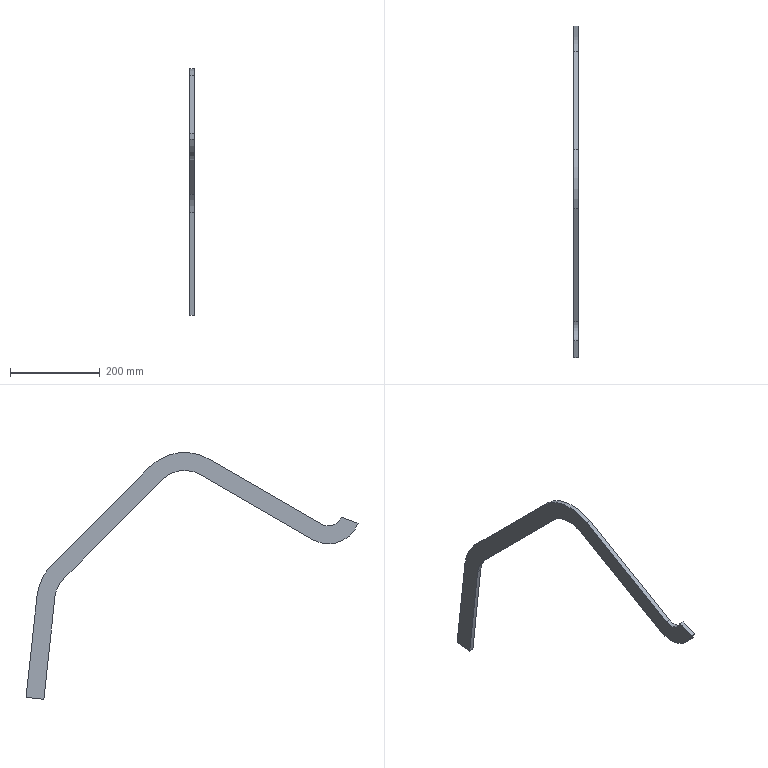Component | SolidWorks | Rebro sipke-3-109 | 1 solid | 16 faces | box 10 x 740.76 x 550.54 mm | volume 438581 mm3 | plane 10 | cylinder 6 | commonest cylinder face diameters 140 x3 220 x2 60 x1
build123d program:
from build123d import *

# Parameters (mm, degrees)
BOSS_EXTRUDE1_DEPTH = 10


with BuildPart() as part:
    # Sketch1 → Boss-Extrude1 (new body)
    with BuildSketch(Plane.XY):
        with BuildLine():
            Line((626.269, -76.361), (701.294, 203.766))
            ThreePointArc((701.294, 203.766), (739.32, 249.094), (798.487, 249.101))
            Line((798.487, 249.101), (781.586, 212.847))
            ThreePointArc((781.586, 212.847), (756.229, 212.844), (739.932, 193.418))
            Line((739.932, 193.418), (664.907, -86.71))
            ThreePointArc((664.907, -86.71), (625.621, -145.517), (558.652, -168.252))
            Line((558.652, -168.252), (248.065, -168.252))
            ThreePointArc((248.065, -168.252), (211.537, -162.01), (179.154, -143.991))
            Line((179.154, -143.991), (0, 0))
            Line((0, 0), (25.059, 31.178))
            Line((25.059, 31.178), (204.213, -112.813))
            ThreePointArc((204.213, -112.813), (224.82, -124.279), (248.065, -128.252))
            Line((248.065, -128.252), (558.652, -128.252))
            ThreePointArc((558.652, -128.252), (601.269, -113.784), (626.269, -76.361))
        make_face()
    extrude(amount=-BOSS_EXTRUDE1_DEPTH)


solid = part.part

# Placed as in the assembly
solid = solid.moved(Location((-91.6, -141.455, -674.126), (-135, 90, 0)))
STEP:
#1=COLOUR_RGB('',0.7922,0.8196,0.9333);
#2=FILL_AREA_STYLE_COLOUR('',#1);
#3=FILL_AREA_STYLE('',(#2));
#4=SURFACE_STYLE_FILL_AREA(#3);
#5=SURFACE_SIDE_STYLE('',(#4));
#6=SURFACE_STYLE_USAGE(.BOTH.,#5);
#7=PRESENTATION_STYLE_ASSIGNMENT((#6));
#8=CARTESIAN_POINT('',(-3.606,-34.733,-11.246));
#9=VERTEX_POINT('',#8);
#10=CARTESIAN_POINT('',(-3.606,-30.765,-12.69));
#11=VERTEX_POINT('',#10);
#12=CARTESIAN_POINT('',(-3.606,-32.143,-10.303));
#13=DIRECTION('',(1.,-0.,-0.));
#14=DIRECTION('',(0.,-0.7071,0.7071));
#15=AXIS2_PLACEMENT_3D('',#12,#13,#14);
#16=CIRCLE('',#15,2.756);
#17=EDGE_CURVE('',#9,#11,#16,.T.);
#18=ORIENTED_EDGE('',*,*,#17,.F.);
#19=CARTESIAN_POINT('',(-4.,-34.733,-11.246));
#20=VERTEX_POINT('',#19);
#21=CARTESIAN_POINT('',(-4.,-34.733,-11.246));
#22=DIRECTION('',(1.,-0.,-0.));
#23=VECTOR('',#22,39.37);
#24=LINE('',#21,#23);
#25=EDGE_CURVE('',#20,#9,#24,.T.);
#26=ORIENTED_EDGE('',*,*,#25,.F.);
#27=CARTESIAN_POINT('',(-4.,-30.765,-12.69));
#28=VERTEX_POINT('',#27);
#29=CARTESIAN_POINT('',(-4.,-32.143,-10.303));
#30=DIRECTION('',(1.,-0.,-0.));
#31=DIRECTION('',(0.,-0.7071,0.7071));
#32=AXIS2_PLACEMENT_3D('',#29,#30,#31);
#33=CIRCLE('',#32,2.756);
#34=EDGE_CURVE('',#20,#28,#33,.T.);
#35=ORIENTED_EDGE('',*,*,#34,.T.);
#36=CARTESIAN_POINT('',(-4.,-30.765,-12.69));
#37=DIRECTION('',(1.,-0.,-0.));
#38=VECTOR('',#37,39.37);
#39=LINE('',#36,#38);
#40=EDGE_CURVE('',#28,#11,#39,.T.);
#41=ORIENTED_EDGE('',*,*,#40,.T.);
#42=EDGE_LOOP('',(#18,#26,#35,#41));
#43=FACE_OUTER_BOUND('',#42,.T.);
#44=CARTESIAN_POINT('',(-4.,-32.143,-10.303));
#45=DIRECTION('',(1.,-0.,-0.));
#46=DIRECTION('',(0.,-0.7071,0.7071));
#47=AXIS2_PLACEMENT_3D('',#44,#45,#46);
#48=CYLINDRICAL_SURFACE('',#47,2.756);
#49=ADVANCED_FACE('',(#43),#48,.T.);
#50=CARTESIAN_POINT('',(-3.606,-33.253,-10.707));
#51=VERTEX_POINT('',#50);
#52=CARTESIAN_POINT('',(-3.606,-33.253,-10.707));
#53=DIRECTION('',(-0.,-0.9397,-0.3421));
#54=VECTOR('',#53,39.37);
#55=LINE('',#52,#54);
#56=EDGE_CURVE('',#51,#9,#55,.T.);
#57=ORIENTED_EDGE('',*,*,#56,.F.);
#58=CARTESIAN_POINT('',(-4.,-33.253,-10.707));
#59=VERTEX_POINT('',#58);
#60=CARTESIAN_POINT('',(-4.,-33.253,-10.707));
#61=DIRECTION('',(1.,-0.,-0.));
#62=VECTOR('',#61,39.37);
#63=LINE('',#60,#62);
#64=EDGE_CURVE('',#59,#51,#63,.T.);
#65=ORIENTED_EDGE('',*,*,#64,.F.);
#66=CARTESIAN_POINT('',(-4.,-33.253,-10.707));
#67=DIRECTION('',(-0.,-0.9397,-0.3421));
#68=VECTOR('',#67,39.37);
#69=LINE('',#66,#68);
#70=EDGE_CURVE('',#59,#20,#69,.T.);
#71=ORIENTED_EDGE('',*,*,#70,.T.);
#72=ORIENTED_EDGE('',*,*,#25,.T.);
#73=EDGE_LOOP('',(#57,#65,#71,#72));
#74=FACE_OUTER_BOUND('',#73,.T.);
#75=CARTESIAN_POINT('',(-4.,-33.253,-10.707));
#76=DIRECTION('',(0.,-0.3421,0.9397));
#77=DIRECTION('',(-0.,-0.9397,-0.3421));
#78=AXIS2_PLACEMENT_3D('',#75,#76,#77);
#79=PLANE('',#78);
#80=ADVANCED_FACE('',(#74),#79,.T.);
#81=CARTESIAN_POINT('',(-3.606,-31.552,-11.326));
#82=VERTEX_POINT('',#81);
#83=CARTESIAN_POINT('',(-3.606,-32.143,-10.303));
#84=DIRECTION('',(-1.,0.,0.));
#85=DIRECTION('',(0.,-0.7071,0.7071));
#86=AXIS2_PLACEMENT_3D('',#83,#84,#85);
#87=CIRCLE('',#86,1.181);
#88=EDGE_CURVE('',#82,#51,#87,.T.);
#89=ORIENTED_EDGE('',*,*,#88,.F.);
#90=CARTESIAN_POINT('',(-4.,-31.552,-11.326));
#91=VERTEX_POINT('',#90);
#92=CARTESIAN_POINT('',(-4.,-31.552,-11.326));
#93=DIRECTION('',(1.,-0.,-0.));
#94=VECTOR('',#93,39.37);
#95=LINE('',#92,#94);
#96=EDGE_CURVE('',#91,#82,#95,.T.);
#97=ORIENTED_EDGE('',*,*,#96,.F.);
#98=CARTESIAN_POINT('',(-4.,-32.143,-10.303));
#99=DIRECTION('',(-1.,0.,0.));
#100=DIRECTION('',(0.,-0.7071,0.7071));
#101=AXIS2_PLACEMENT_3D('',#98,#99,#100);
#102=CIRCLE('',#101,1.181);
#103=EDGE_CURVE('',#91,#59,#102,.T.);
#104=ORIENTED_EDGE('',*,*,#103,.T.);
#105=ORIENTED_EDGE('',*,*,#64,.T.);
#106=EDGE_LOOP('',(#89,#97,#104,#105));
#107=FACE_OUTER_BOUND('',#106,.T.);
#108=CARTESIAN_POINT('',(-4.,-32.143,-10.303));
#109=DIRECTION('',(1.,-0.,-0.));
#110=DIRECTION('',(0.,-0.7071,0.7071));
#111=AXIS2_PLACEMENT_3D('',#108,#109,#110);
#112=CYLINDRICAL_SURFACE('',#111,1.181);
#113=ADVANCED_FACE('',(#107),#112,.F.);
#114=CARTESIAN_POINT('',(-3.606,-21.665,-5.616));
#115=VERTEX_POINT('',#114);
#116=CARTESIAN_POINT('',(-3.606,-21.665,-5.616));
#117=DIRECTION('',(-0.,-0.866,-0.5001));
#118=VECTOR('',#117,39.37);
#119=LINE('',#116,#118);
#120=EDGE_CURVE('',#115,#82,#119,.T.);
#121=ORIENTED_EDGE('',*,*,#120,.F.);
#122=CARTESIAN_POINT('',(-4.,-21.665,-5.616));
#123=VERTEX_POINT('',#122);
#124=CARTESIAN_POINT('',(-4.,-21.665,-5.616));
#125=DIRECTION('',(1.,-0.,-0.));
#126=VECTOR('',#125,39.37);
#127=LINE('',#124,#126);
#128=EDGE_CURVE('',#123,#115,#127,.T.);
#129=ORIENTED_EDGE('',*,*,#128,.F.);
#130=CARTESIAN_POINT('',(-4.,-21.665,-5.616));
#131=DIRECTION('',(-0.,-0.866,-0.5001));
#132=VECTOR('',#131,39.37);
#133=LINE('',#130,#132);
#134=EDGE_CURVE('',#123,#91,#133,.T.);
#135=ORIENTED_EDGE('',*,*,#134,.T.);
#136=ORIENTED_EDGE('',*,*,#96,.T.);
#137=EDGE_LOOP('',(#121,#129,#135,#136));
#138=FACE_OUTER_BOUND('',#137,.T.);
#139=CARTESIAN_POINT('',(-4.,-21.665,-5.616));
#140=DIRECTION('',(0.,-0.5001,0.866));
#141=DIRECTION('',(-0.,-0.866,-0.5001));
#142=AXIS2_PLACEMENT_3D('',#139,#140,#141);
#143=PLANE('',#142);
#144=ADVANCED_FACE('',(#138),#143,.T.);
#145=CARTESIAN_POINT('',(-3.606,-16.437,-6.304));
#146=VERTEX_POINT('',#145);
#147=CARTESIAN_POINT('',(-3.606,-19.5,-9.366));
#148=DIRECTION('',(1.,-0.,-0.));
#149=DIRECTION('',(0.,-0.7071,0.7071));
#150=AXIS2_PLACEMENT_3D('',#147,#148,#149);
#151=CIRCLE('',#150,4.331);
#152=EDGE_CURVE('',#146,#115,#151,.T.);
#153=ORIENTED_EDGE('',*,*,#152,.F.);
#154=CARTESIAN_POINT('',(-4.,-16.437,-6.304));
#155=VERTEX_POINT('',#154);
#156=CARTESIAN_POINT('',(-4.,-16.437,-6.304));
#157=DIRECTION('',(1.,-0.,-0.));
#158=VECTOR('',#157,39.37);
#159=LINE('',#156,#158);
#160=EDGE_CURVE('',#155,#146,#159,.T.);
#161=ORIENTED_EDGE('',*,*,#160,.F.);
#162=CARTESIAN_POINT('',(-4.,-19.5,-9.366));
#163=DIRECTION('',(1.,-0.,-0.));
#164=DIRECTION('',(0.,-0.7071,0.7071));
#165=AXIS2_PLACEMENT_3D('',#162,#163,#164);
#166=CIRCLE('',#165,4.331);
#167=EDGE_CURVE('',#155,#123,#166,.T.);
#168=ORIENTED_EDGE('',*,*,#167,.T.);
#169=ORIENTED_EDGE('',*,*,#128,.T.);
#170=EDGE_LOOP('',(#153,#161,#168,#169));
#171=FACE_OUTER_BOUND('',#170,.T.);
#172=CARTESIAN_POINT('',(-4.,-19.5,-9.366));
#173=DIRECTION('',(1.,-0.,-0.));
#174=DIRECTION('',(0.,-0.7071,0.7071));
#175=AXIS2_PLACEMENT_3D('',#172,#173,#174);
#176=CYLINDRICAL_SURFACE('',#175,4.331);
#177=ADVANCED_FACE('',(#171),#176,.T.);
#178=CARTESIAN_POINT('',(-3.606,-7.791,-14.951));
#179=VERTEX_POINT('',#178);
#180=CARTESIAN_POINT('',(-3.606,-7.791,-14.951));
#181=DIRECTION('',(0.,-0.7071,0.7071));
#182=VECTOR('',#181,39.37);
#183=LINE('',#180,#182);
#184=EDGE_CURVE('',#179,#146,#183,.T.);
#185=ORIENTED_EDGE('',*,*,#184,.F.);
#186=CARTESIAN_POINT('',(-4.,-7.791,-14.951));
#187=VERTEX_POINT('',#186);
#188=CARTESIAN_POINT('',(-4.,-7.791,-14.951));
#189=DIRECTION('',(1.,-0.,-0.));
#190=VECTOR('',#189,39.37);
#191=LINE('',#188,#190);
#192=EDGE_CURVE('',#187,#179,#191,.T.);
#193=ORIENTED_EDGE('',*,*,#192,.F.);
#194=CARTESIAN_POINT('',(-4.,-7.791,-14.951));
#195=DIRECTION('',(0.,-0.7071,0.7071));
#196=VECTOR('',#195,39.37);
#197=LINE('',#194,#196);
#198=EDGE_CURVE('',#187,#155,#197,.T.);
#199=ORIENTED_EDGE('',*,*,#198,.T.);
#200=ORIENTED_EDGE('',*,*,#160,.T.);
#201=EDGE_LOOP('',(#185,#193,#199,#200));
#202=FACE_OUTER_BOUND('',#201,.T.);
#203=CARTESIAN_POINT('',(-4.,-7.791,-14.951));
#204=DIRECTION('',(0.,0.7071,0.7071));
#205=DIRECTION('',(-1.,0.,0.));
#206=AXIS2_PLACEMENT_3D('',#203,#204,#205);
#207=PLANE('',#206);
#208=ADVANCED_FACE('',(#202),#207,.T.);
#209=CARTESIAN_POINT('',(-3.606,-6.548,-17.544));
#210=VERTEX_POINT('',#209);
#211=CARTESIAN_POINT('',(-3.606,-10.853,-18.013));
#212=DIRECTION('',(1.,-0.,-0.));
#213=DIRECTION('',(0.,-0.7071,0.7071));
#214=AXIS2_PLACEMENT_3D('',#211,#212,#213);
#215=CIRCLE('',#214,4.331);
#216=EDGE_CURVE('',#210,#179,#215,.T.);
#217=ORIENTED_EDGE('',*,*,#216,.F.);
#218=CARTESIAN_POINT('',(-4.,-6.548,-17.544));
#219=VERTEX_POINT('',#218);
#220=CARTESIAN_POINT('',(-4.,-6.548,-17.544));
#221=DIRECTION('',(1.,-0.,-0.));
#222=VECTOR('',#221,39.37);
#223=LINE('',#220,#222);
#224=EDGE_CURVE('',#219,#210,#223,.T.);
#225=ORIENTED_EDGE('',*,*,#224,.F.);
#226=CARTESIAN_POINT('',(-4.,-10.853,-18.013));
#227=DIRECTION('',(1.,-0.,-0.));
#228=DIRECTION('',(0.,-0.7071,0.7071));
#229=AXIS2_PLACEMENT_3D('',#226,#227,#228);
#230=CIRCLE('',#229,4.331);
#231=EDGE_CURVE('',#219,#187,#230,.T.);
#232=ORIENTED_EDGE('',*,*,#231,.T.);
#233=ORIENTED_EDGE('',*,*,#192,.T.);
#234=EDGE_LOOP('',(#217,#225,#232,#233));
#235=FACE_OUTER_BOUND('',#234,.T.);
#236=CARTESIAN_POINT('',(-4.,-10.853,-18.013));
#237=DIRECTION('',(1.,-0.,-0.));
#238=DIRECTION('',(0.,-0.7071,0.7071));
#239=AXIS2_PLACEMENT_3D('',#236,#237,#238);
#240=CYLINDRICAL_SURFACE('',#239,4.331);
#241=ADVANCED_FACE('',(#235),#240,.T.);
#242=CARTESIAN_POINT('',(-3.606,-5.569,-26.54));
#243=VERTEX_POINT('',#242);
#244=CARTESIAN_POINT('',(-3.606,-5.569,-26.54));
#245=DIRECTION('',(0.,-0.1082,0.9941));
#246=VECTOR('',#245,39.37);
#247=LINE('',#244,#246);
#248=EDGE_CURVE('',#243,#210,#247,.T.);
#249=ORIENTED_EDGE('',*,*,#248,.F.);
#250=CARTESIAN_POINT('',(-4.,-5.569,-26.54));
#251=VERTEX_POINT('',#250);
#252=CARTESIAN_POINT('',(-4.,-5.569,-26.54));
#253=DIRECTION('',(1.,-0.,-0.));
#254=VECTOR('',#253,39.37);
#255=LINE('',#252,#254);
#256=EDGE_CURVE('',#251,#243,#255,.T.);
#257=ORIENTED_EDGE('',*,*,#256,.F.);
#258=CARTESIAN_POINT('',(-4.,-5.569,-26.54));
#259=DIRECTION('',(0.,-0.1082,0.9941));
#260=VECTOR('',#259,39.37);
#261=LINE('',#258,#260);
#262=EDGE_CURVE('',#251,#219,#261,.T.);
#263=ORIENTED_EDGE('',*,*,#262,.T.);
#264=ORIENTED_EDGE('',*,*,#224,.T.);
#265=EDGE_LOOP('',(#249,#257,#263,#264));
#266=FACE_OUTER_BOUND('',#265,.T.);
#267=CARTESIAN_POINT('',(-4.,-5.569,-26.54));
#268=DIRECTION('',(0.,0.9941,0.1082));
#269=DIRECTION('',(0.,-0.1082,0.9941));
#270=AXIS2_PLACEMENT_3D('',#267,#268,#269);
#271=PLANE('',#270);
#272=ADVANCED_FACE('',(#266),#271,.T.);
#273=CARTESIAN_POINT('',(-3.606,-7.135,-26.711));
#274=VERTEX_POINT('',#273);
#275=CARTESIAN_POINT('',(-3.606,-5.569,-26.54));
#276=DIRECTION('',(0.,0.9941,0.1082));
#277=VECTOR('',#276,39.37);
#278=LINE('',#275,#277);
#279=EDGE_CURVE('',#274,#243,#278,.T.);
#280=ORIENTED_EDGE('',*,*,#279,.F.);
#281=CARTESIAN_POINT('',(-4.,-7.135,-26.711));
#282=VERTEX_POINT('',#281);
#283=CARTESIAN_POINT('',(-4.,-7.135,-26.711));
#284=DIRECTION('',(1.,-0.,-0.));
#285=VECTOR('',#284,39.37);
#286=LINE('',#283,#285);
#287=EDGE_CURVE('',#282,#274,#286,.T.);
#288=ORIENTED_EDGE('',*,*,#287,.F.);
#289=CARTESIAN_POINT('',(-4.,-5.569,-26.54));
#290=DIRECTION('',(0.,0.9941,0.1082));
#291=VECTOR('',#290,39.37);
#292=LINE('',#289,#291);
#293=EDGE_CURVE('',#282,#251,#292,.T.);
#294=ORIENTED_EDGE('',*,*,#293,.T.);
#295=ORIENTED_EDGE('',*,*,#256,.T.);
#296=EDGE_LOOP('',(#280,#288,#294,#295));
#297=FACE_OUTER_BOUND('',#296,.T.);
#298=CARTESIAN_POINT('',(-4.,-5.569,-26.54));
#299=DIRECTION('',(-0.,0.1082,-0.9941));
#300=DIRECTION('',(0.,0.9941,0.1082));
#301=AXIS2_PLACEMENT_3D('',#298,#299,#300);
#302=PLANE('',#301);
#303=ADVANCED_FACE('',(#297),#302,.T.);
#304=CARTESIAN_POINT('',(-3.606,-8.114,-17.715));
#305=VERTEX_POINT('',#304);
#306=CARTESIAN_POINT('',(-3.606,-7.135,-26.711));
#307=DIRECTION('',(-0.,0.1082,-0.9941));
#308=VECTOR('',#307,39.37);
#309=LINE('',#306,#308);
#310=EDGE_CURVE('',#305,#274,#309,.T.);
#311=ORIENTED_EDGE('',*,*,#310,.F.);
#312=CARTESIAN_POINT('',(-4.,-8.114,-17.715));
#313=VERTEX_POINT('',#312);
#314=CARTESIAN_POINT('',(-4.,-8.114,-17.715));
#315=DIRECTION('',(1.,-0.,-0.));
#316=VECTOR('',#315,39.37);
#317=LINE('',#314,#316);
#318=EDGE_CURVE('',#313,#305,#317,.T.);
#319=ORIENTED_EDGE('',*,*,#318,.F.);
#320=CARTESIAN_POINT('',(-4.,-7.135,-26.711));
#321=DIRECTION('',(-0.,0.1082,-0.9941));
#322=VECTOR('',#321,39.37);
#323=LINE('',#320,#322);
#324=EDGE_CURVE('',#313,#282,#323,.T.);
#325=ORIENTED_EDGE('',*,*,#324,.T.);
#326=ORIENTED_EDGE('',*,*,#287,.T.);
#327=EDGE_LOOP('',(#311,#319,#325,#326));
#328=FACE_OUTER_BOUND('',#327,.T.);
#329=CARTESIAN_POINT('',(-4.,-7.135,-26.711));
#330=DIRECTION('',(-0.,-0.9941,-0.1082));
#331=DIRECTION('',(-0.,0.1082,-0.9941));
#332=AXIS2_PLACEMENT_3D('',#329,#330,#331);
#333=PLANE('',#332);
#334=ADVANCED_FACE('',(#328),#333,.T.);
#335=CARTESIAN_POINT('',(-3.606,-8.905,-16.064));
#336=VERTEX_POINT('',#335);
#337=CARTESIAN_POINT('',(-3.606,-10.853,-18.013));
#338=DIRECTION('',(-1.,0.,0.));
#339=DIRECTION('',(0.,-0.7071,0.7071));
#340=AXIS2_PLACEMENT_3D('',#337,#338,#339);
#341=CIRCLE('',#340,2.756);
#342=EDGE_CURVE('',#336,#305,#341,.T.);
#343=ORIENTED_EDGE('',*,*,#342,.F.);
#344=CARTESIAN_POINT('',(-4.,-8.905,-16.064));
#345=VERTEX_POINT('',#344);
#346=CARTESIAN_POINT('',(-4.,-8.905,-16.064));
#347=DIRECTION('',(1.,-0.,-0.));
#348=VECTOR('',#347,39.37);
#349=LINE('',#346,#348);
#350=EDGE_CURVE('',#345,#336,#349,.T.);
#351=ORIENTED_EDGE('',*,*,#350,.F.);
#352=CARTESIAN_POINT('',(-4.,-10.853,-18.013));
#353=DIRECTION('',(-1.,0.,0.));
#354=DIRECTION('',(0.,-0.7071,0.7071));
#355=AXIS2_PLACEMENT_3D('',#352,#353,#354);
#356=CIRCLE('',#355,2.756);
#357=EDGE_CURVE('',#345,#313,#356,.T.);
#358=ORIENTED_EDGE('',*,*,#357,.T.);
#359=ORIENTED_EDGE('',*,*,#318,.T.);
#360=EDGE_LOOP('',(#343,#351,#358,#359));
#361=FACE_OUTER_BOUND('',#360,.T.);
#362=CARTESIAN_POINT('',(-4.,-10.853,-18.013));
#363=DIRECTION('',(1.,-0.,-0.));
#364=DIRECTION('',(0.,-0.7071,0.7071));
#365=AXIS2_PLACEMENT_3D('',#362,#363,#364);
#366=CYLINDRICAL_SURFACE('',#365,2.756);
#367=ADVANCED_FACE('',(#361),#366,.F.);
#368=CARTESIAN_POINT('',(-3.606,-17.551,-7.418));
#369=VERTEX_POINT('',#368);
#370=CARTESIAN_POINT('',(-3.606,-8.905,-16.064));
#371=DIRECTION('',(-0.,0.7071,-0.7071));
#372=VECTOR('',#371,39.37);
#373=LINE('',#370,#372);
#374=EDGE_CURVE('',#369,#336,#373,.T.);
#375=ORIENTED_EDGE('',*,*,#374,.F.);
#376=CARTESIAN_POINT('',(-4.,-17.551,-7.418));
#377=VERTEX_POINT('',#376);
#378=CARTESIAN_POINT('',(-4.,-17.551,-7.418));
#379=DIRECTION('',(1.,-0.,-0.));
#380=VECTOR('',#379,39.37);
#381=LINE('',#378,#380);
#382=EDGE_CURVE('',#377,#369,#381,.T.);
#383=ORIENTED_EDGE('',*,*,#382,.F.);
#384=CARTESIAN_POINT('',(-4.,-8.905,-16.064));
#385=DIRECTION('',(-0.,0.7071,-0.7071));
#386=VECTOR('',#385,39.37);
#387=LINE('',#384,#386);
#388=EDGE_CURVE('',#377,#345,#387,.T.);
#389=ORIENTED_EDGE('',*,*,#388,.T.);
#390=ORIENTED_EDGE('',*,*,#350,.T.);
#391=EDGE_LOOP('',(#375,#383,#389,#390));
#392=FACE_OUTER_BOUND('',#391,.T.);
#393=CARTESIAN_POINT('',(-4.,-8.905,-16.064));
#394=DIRECTION('',(-0.,-0.7071,-0.7071));
#395=DIRECTION('',(1.,-0.,-0.));
#396=AXIS2_PLACEMENT_3D('',#393,#394,#395);
#397=PLANE('',#396);
#398=ADVANCED_FACE('',(#392),#397,.T.);
#399=CARTESIAN_POINT('',(-3.606,-20.878,-6.98));
#400=VERTEX_POINT('',#399);
#401=CARTESIAN_POINT('',(-3.606,-19.5,-9.366));
#402=DIRECTION('',(-1.,0.,0.));
#403=DIRECTION('',(0.,-0.7071,0.7071));
#404=AXIS2_PLACEMENT_3D('',#401,#402,#403);
#405=CIRCLE('',#404,2.756);
#406=EDGE_CURVE('',#400,#369,#405,.T.);
#407=ORIENTED_EDGE('',*,*,#406,.F.);
#408=CARTESIAN_POINT('',(-4.,-20.878,-6.98));
#409=VERTEX_POINT('',#408);
#410=CARTESIAN_POINT('',(-4.,-20.878,-6.98));
#411=DIRECTION('',(1.,-0.,-0.));
#412=VECTOR('',#411,39.37);
#413=LINE('',#410,#412);
#414=EDGE_CURVE('',#409,#400,#413,.T.);
#415=ORIENTED_EDGE('',*,*,#414,.F.);
#416=CARTESIAN_POINT('',(-4.,-19.5,-9.366));
#417=DIRECTION('',(-1.,0.,0.));
#418=DIRECTION('',(0.,-0.7071,0.7071));
#419=AXIS2_PLACEMENT_3D('',#416,#417,#418);
#420=CIRCLE('',#419,2.756);
#421=EDGE_CURVE('',#409,#377,#420,.T.);
#422=ORIENTED_EDGE('',*,*,#421,.T.);
#423=ORIENTED_EDGE('',*,*,#382,.T.);
#424=EDGE_LOOP('',(#407,#415,#422,#423));
#425=FACE_OUTER_BOUND('',#424,.T.);
#426=CARTESIAN_POINT('',(-4.,-19.5,-9.366));
#427=DIRECTION('',(1.,-0.,-0.));
#428=DIRECTION('',(0.,-0.7071,0.7071));
#429=AXIS2_PLACEMENT_3D('',#426,#427,#428);
#430=CYLINDRICAL_SURFACE('',#429,2.756);
#431=ADVANCED_FACE('',(#425),#430,.F.);
#432=CARTESIAN_POINT('',(-3.606,-20.878,-6.98));
#433=DIRECTION('',(0.,0.866,0.5001));
#434=VECTOR('',#433,39.37);
#435=LINE('',#432,#434);
#436=EDGE_CURVE('',#11,#400,#435,.T.);
#437=ORIENTED_EDGE('',*,*,#436,.F.);
#438=ORIENTED_EDGE('',*,*,#40,.F.);
#439=CARTESIAN_POINT('',(-4.,-20.878,-6.98));
#440=DIRECTION('',(0.,0.866,0.5001));
#441=VECTOR('',#440,39.37);
#442=LINE('',#439,#441);
#443=EDGE_CURVE('',#28,#409,#442,.T.);
#444=ORIENTED_EDGE('',*,*,#443,.T.);
#445=ORIENTED_EDGE('',*,*,#414,.T.);
#446=EDGE_LOOP('',(#437,#438,#444,#445));
#447=FACE_OUTER_BOUND('',#446,.T.);
#448=CARTESIAN_POINT('',(-4.,-20.878,-6.98));
#449=DIRECTION('',(-0.,0.5001,-0.866));
#450=DIRECTION('',(0.,0.866,0.5001));
#451=AXIS2_PLACEMENT_3D('',#448,#449,#450);
#452=PLANE('',#451);
#453=ADVANCED_FACE('',(#447),#452,.T.);
#454=ORIENTED_EDGE('',*,*,#34,.F.);
#455=ORIENTED_EDGE('',*,*,#70,.F.);
#456=ORIENTED_EDGE('',*,*,#103,.F.);
#457=ORIENTED_EDGE('',*,*,#134,.F.);
#458=ORIENTED_EDGE('',*,*,#167,.F.);
#459=ORIENTED_EDGE('',*,*,#198,.F.);
#460=ORIENTED_EDGE('',*,*,#231,.F.);
#461=ORIENTED_EDGE('',*,*,#262,.F.);
#462=ORIENTED_EDGE('',*,*,#293,.F.);
#463=ORIENTED_EDGE('',*,*,#324,.F.);
#464=ORIENTED_EDGE('',*,*,#357,.F.);
#465=ORIENTED_EDGE('',*,*,#388,.F.);
#466=ORIENTED_EDGE('',*,*,#421,.F.);
#467=ORIENTED_EDGE('',*,*,#443,.F.);
#468=EDGE_LOOP('',(#454,#455,#456,#457,#458,#459,#460,#461,#462,#463,#464,#465,#466,#467));
#469=FACE_OUTER_BOUND('',#468,.T.);
#470=CARTESIAN_POINT('',(-4.,-32.143,-10.303));
#471=DIRECTION('',(1.,0.,-0.));
#472=DIRECTION('',(0.,-0.7071,0.7071));
#473=AXIS2_PLACEMENT_3D('',#470,#471,#472);
#474=PLANE('',#473);
#475=ADVANCED_FACE('',(#469),#474,.F.);
#476=ORIENTED_EDGE('',*,*,#17,.T.);
#477=ORIENTED_EDGE('',*,*,#436,.T.);
#478=ORIENTED_EDGE('',*,*,#406,.T.);
#479=ORIENTED_EDGE('',*,*,#374,.T.);
#480=ORIENTED_EDGE('',*,*,#342,.T.);
#481=ORIENTED_EDGE('',*,*,#310,.T.);
#482=ORIENTED_EDGE('',*,*,#279,.T.);
#483=ORIENTED_EDGE('',*,*,#248,.T.);
#484=ORIENTED_EDGE('',*,*,#216,.T.);
#485=ORIENTED_EDGE('',*,*,#184,.T.);
#486=ORIENTED_EDGE('',*,*,#152,.T.);
#487=ORIENTED_EDGE('',*,*,#120,.T.);
#488=ORIENTED_EDGE('',*,*,#88,.T.);
#489=ORIENTED_EDGE('',*,*,#56,.T.);
#490=EDGE_LOOP('',(#476,#477,#478,#479,#480,#481,#482,#483,#484,#485,#486,#487,#488,#489));
#491=FACE_OUTER_BOUND('',#490,.T.);
#492=CARTESIAN_POINT('',(-3.606,-32.143,-10.303));
#493=DIRECTION('',(1.,0.,-0.));
#494=DIRECTION('',(0.,-0.7071,0.7071));
#495=AXIS2_PLACEMENT_3D('',#492,#493,#494);
#496=PLANE('',#495);
#497=ADVANCED_FACE('',(#491),#496,.T.);
#498=CLOSED_SHELL('',(#49,#80,#113,#144,#177,#208,#241,#272,#303,#334,#367,#398,#431,#453,#475,#497));
#499=MANIFOLD_SOLID_BREP('',#498);
#500=STYLED_ITEM('',(#7),#499);
#501=PRESENTATION_LAYER_ASSIGNMENT('','',(#500));
#502=(LENGTH_UNIT()NAMED_UNIT(*)SI_UNIT($,.METRE.));
#503=LENGTH_MEASURE_WITH_UNIT(LENGTH_MEASURE(0.0254),#502);
#504=DIMENSIONAL_EXPONENTS(1.,0.,0.,0.,0.,0.,0.);
#505=(CONVERSION_BASED_UNIT('',#503)LENGTH_UNIT()NAMED_UNIT(#504));
#506=UNCERTAINTY_MEASURE_WITH_UNIT(LENGTH_MEASURE(0.00001),#505,'','');
#507=(NAMED_UNIT(*)PLANE_ANGLE_UNIT()SI_UNIT($,.RADIAN.));
#508=(NAMED_UNIT(*)SI_UNIT($,.STERADIAN.)SOLID_ANGLE_UNIT());
#509=(GEOMETRIC_REPRESENTATION_CONTEXT(3)GLOBAL_UNCERTAINTY_ASSIGNED_CONTEXT((#506))GLOBAL_UNIT_ASSIGNED_CONTEXT((#505,#507,#508))REPRESENTATION_CONTEXT('',''));
#510=MECHANICAL_DESIGN_GEOMETRIC_PRESENTATION_REPRESENTATION('',(#500),#509);
#511=CARTESIAN_POINT('',(0.,0.,0.));
#512=DIRECTION('',(0.,0.,1.));
#513=DIRECTION('',(1.,0.,0.));
#514=AXIS2_PLACEMENT_3D('',#511,#512,#513);
#515=(LENGTH_UNIT()NAMED_UNIT(*)SI_UNIT($,.METRE.));
#516=LENGTH_MEASURE_WITH_UNIT(LENGTH_MEASURE(0.0254),#515);
#517=DIMENSIONAL_EXPONENTS(1.,0.,0.,0.,0.,0.,0.);
#518=(CONVERSION_BASED_UNIT('',#516)LENGTH_UNIT()NAMED_UNIT(#517));
#519=UNCERTAINTY_MEASURE_WITH_UNIT(LENGTH_MEASURE(0.00001),#518,'','');
#520=(NAMED_UNIT(*)PLANE_ANGLE_UNIT()SI_UNIT($,.RADIAN.));
#521=(NAMED_UNIT(*)SI_UNIT($,.STERADIAN.)SOLID_ANGLE_UNIT());
#522=(GEOMETRIC_REPRESENTATION_CONTEXT(3)GLOBAL_UNCERTAINTY_ASSIGNED_CONTEXT((#519))GLOBAL_UNIT_ASSIGNED_CONTEXT((#518,#520,#521))REPRESENTATION_CONTEXT('',''));
#523=ADVANCED_BREP_SHAPE_REPRESENTATION('',(#499,#514),#522);